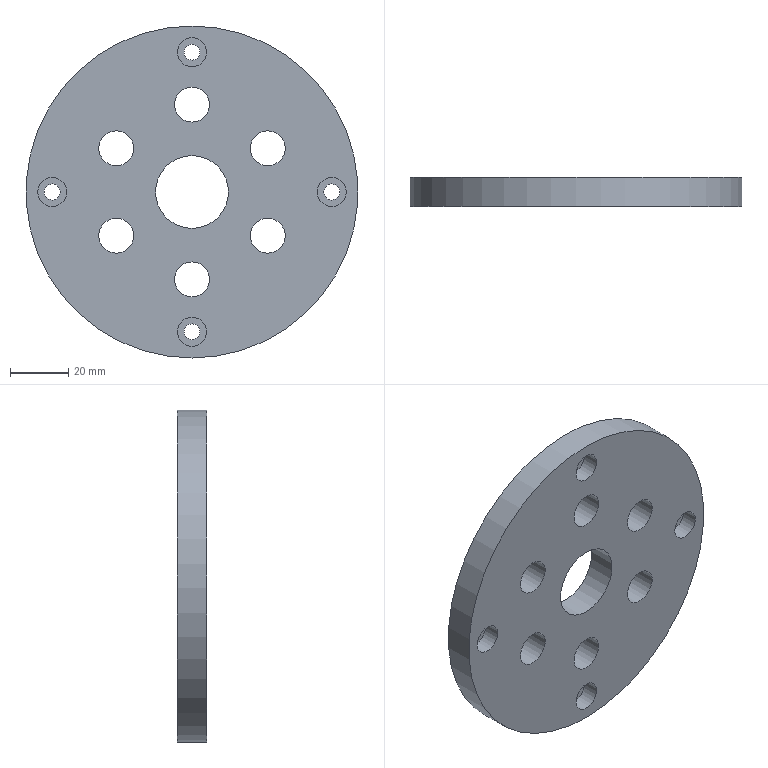Component | NX | PORT_PLATE | 1 solid | 22 faces | volume 88155 mm3 | cylinder 16 | plane 6 | commonest cylinder face diameters 12 x6 5.5 x4 10 x4 25 x1 114 x1